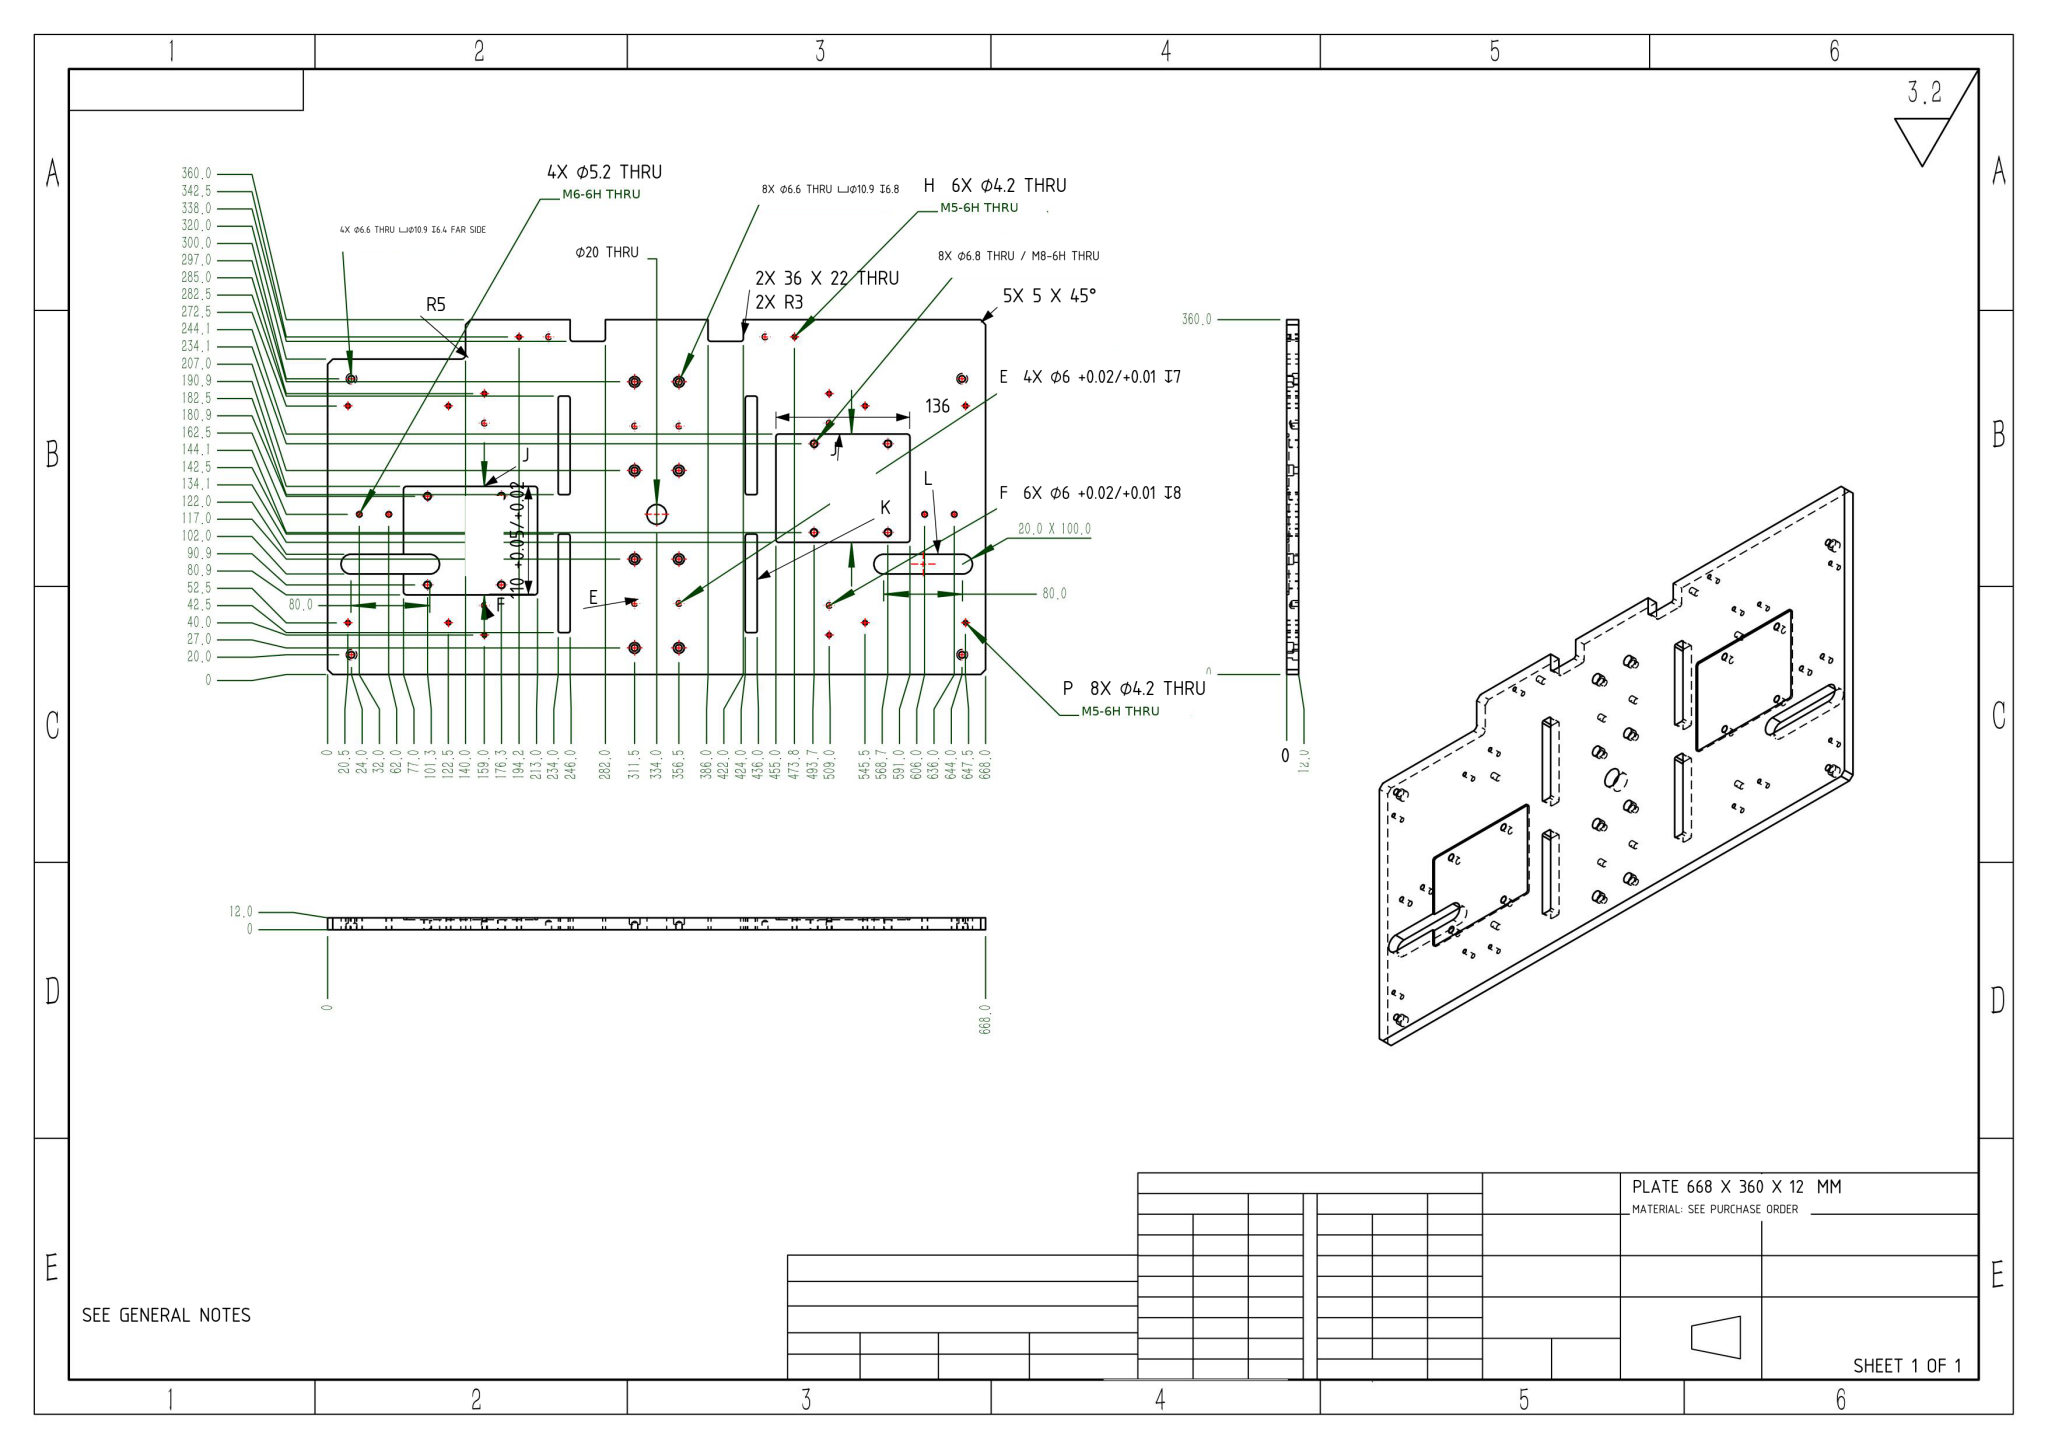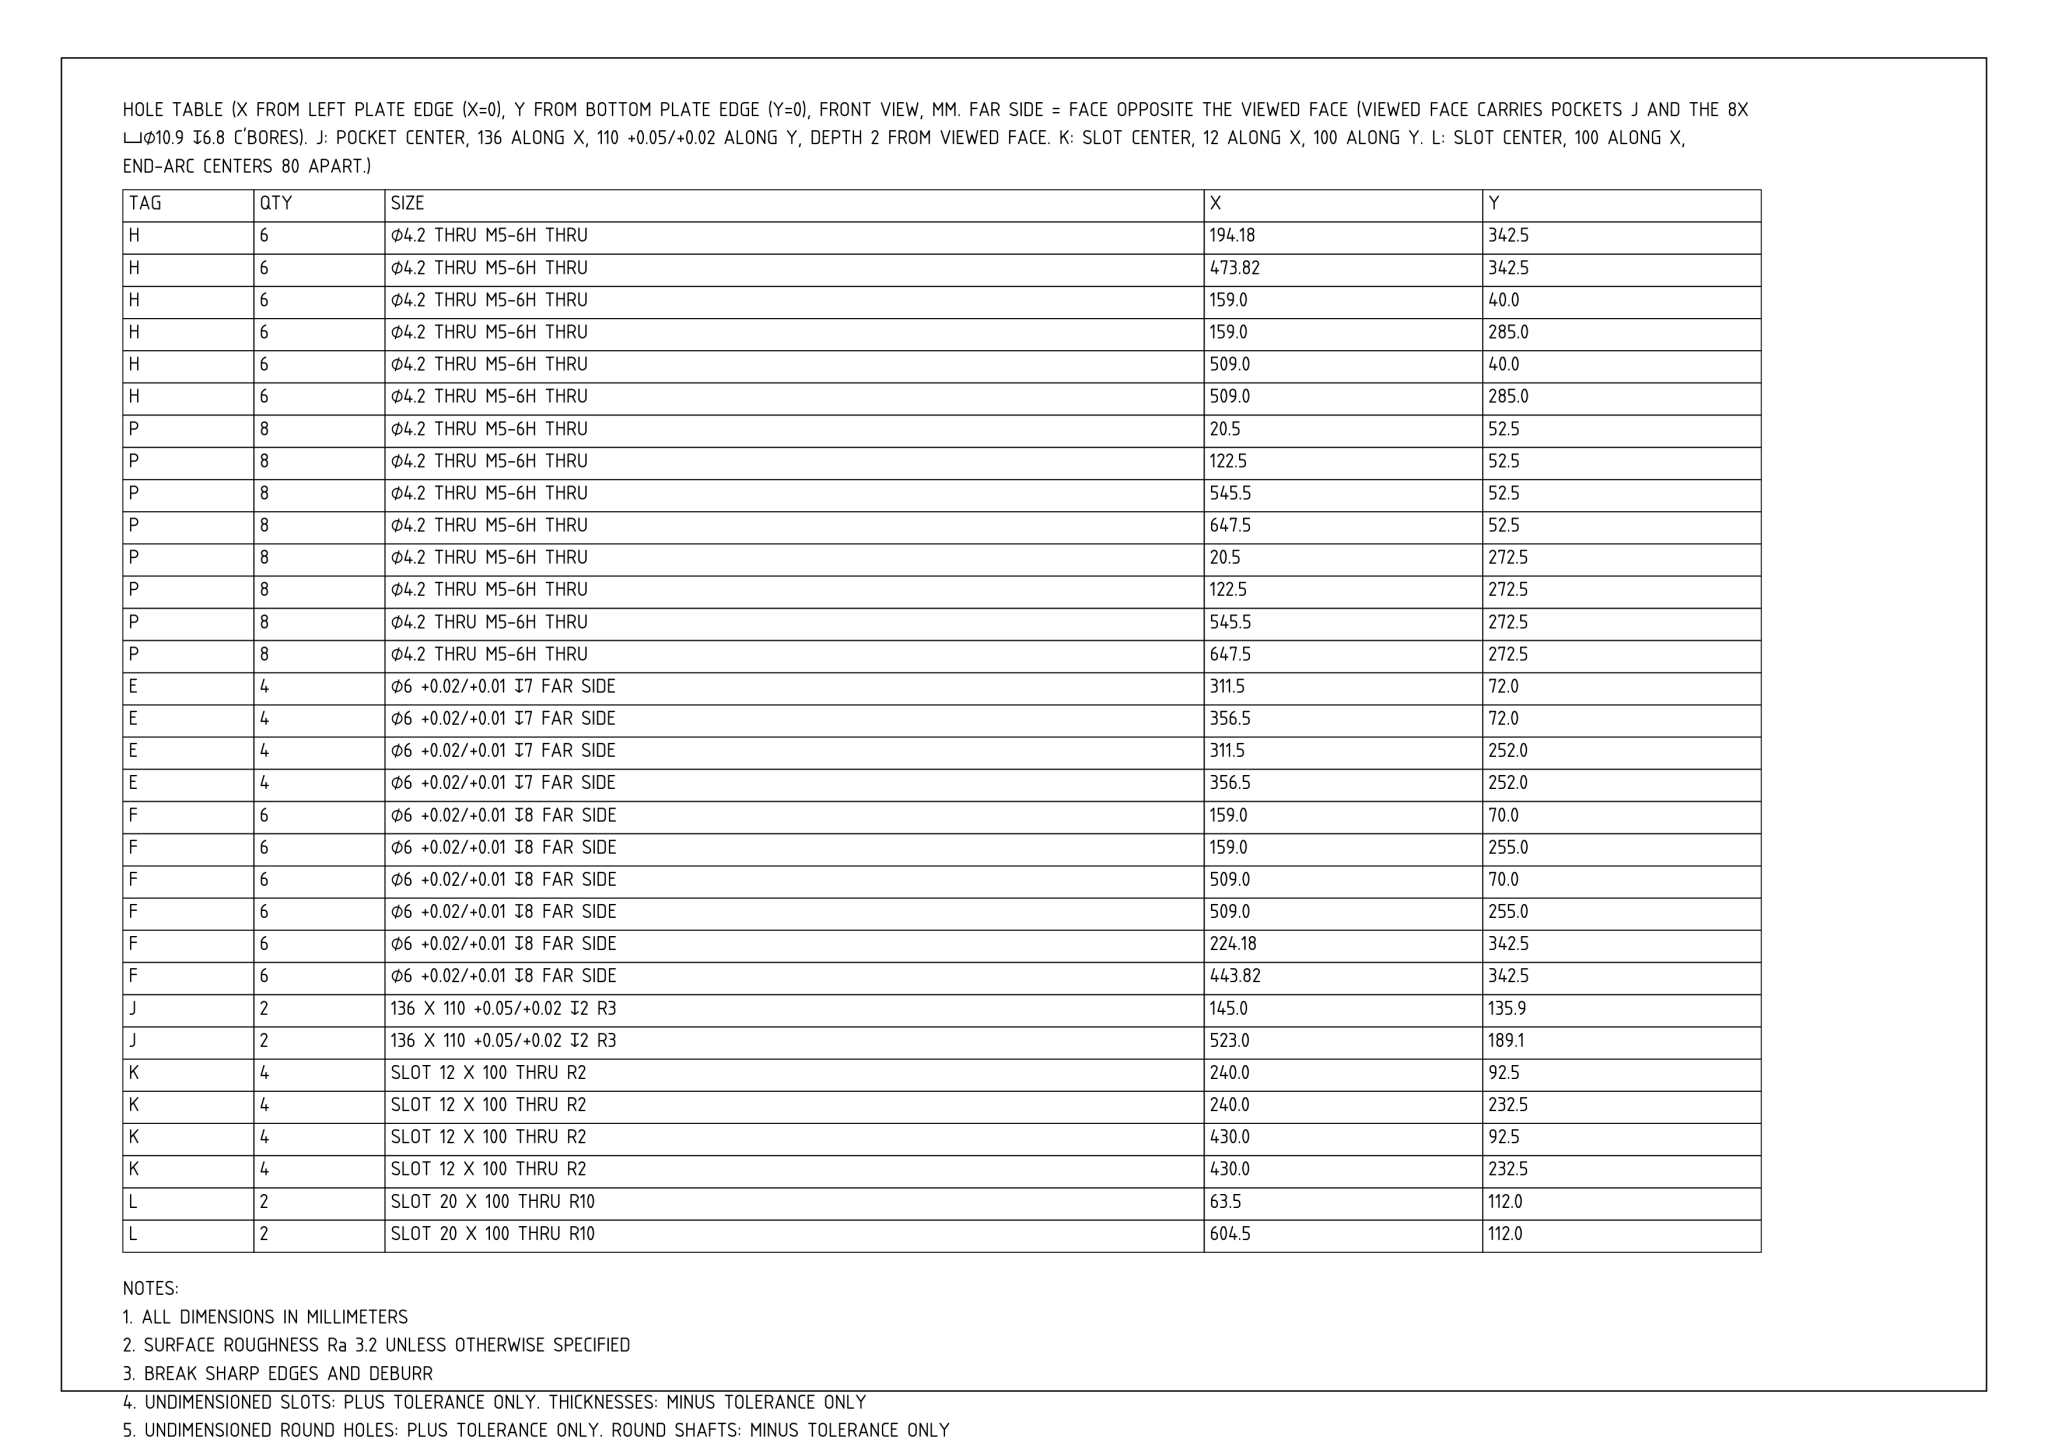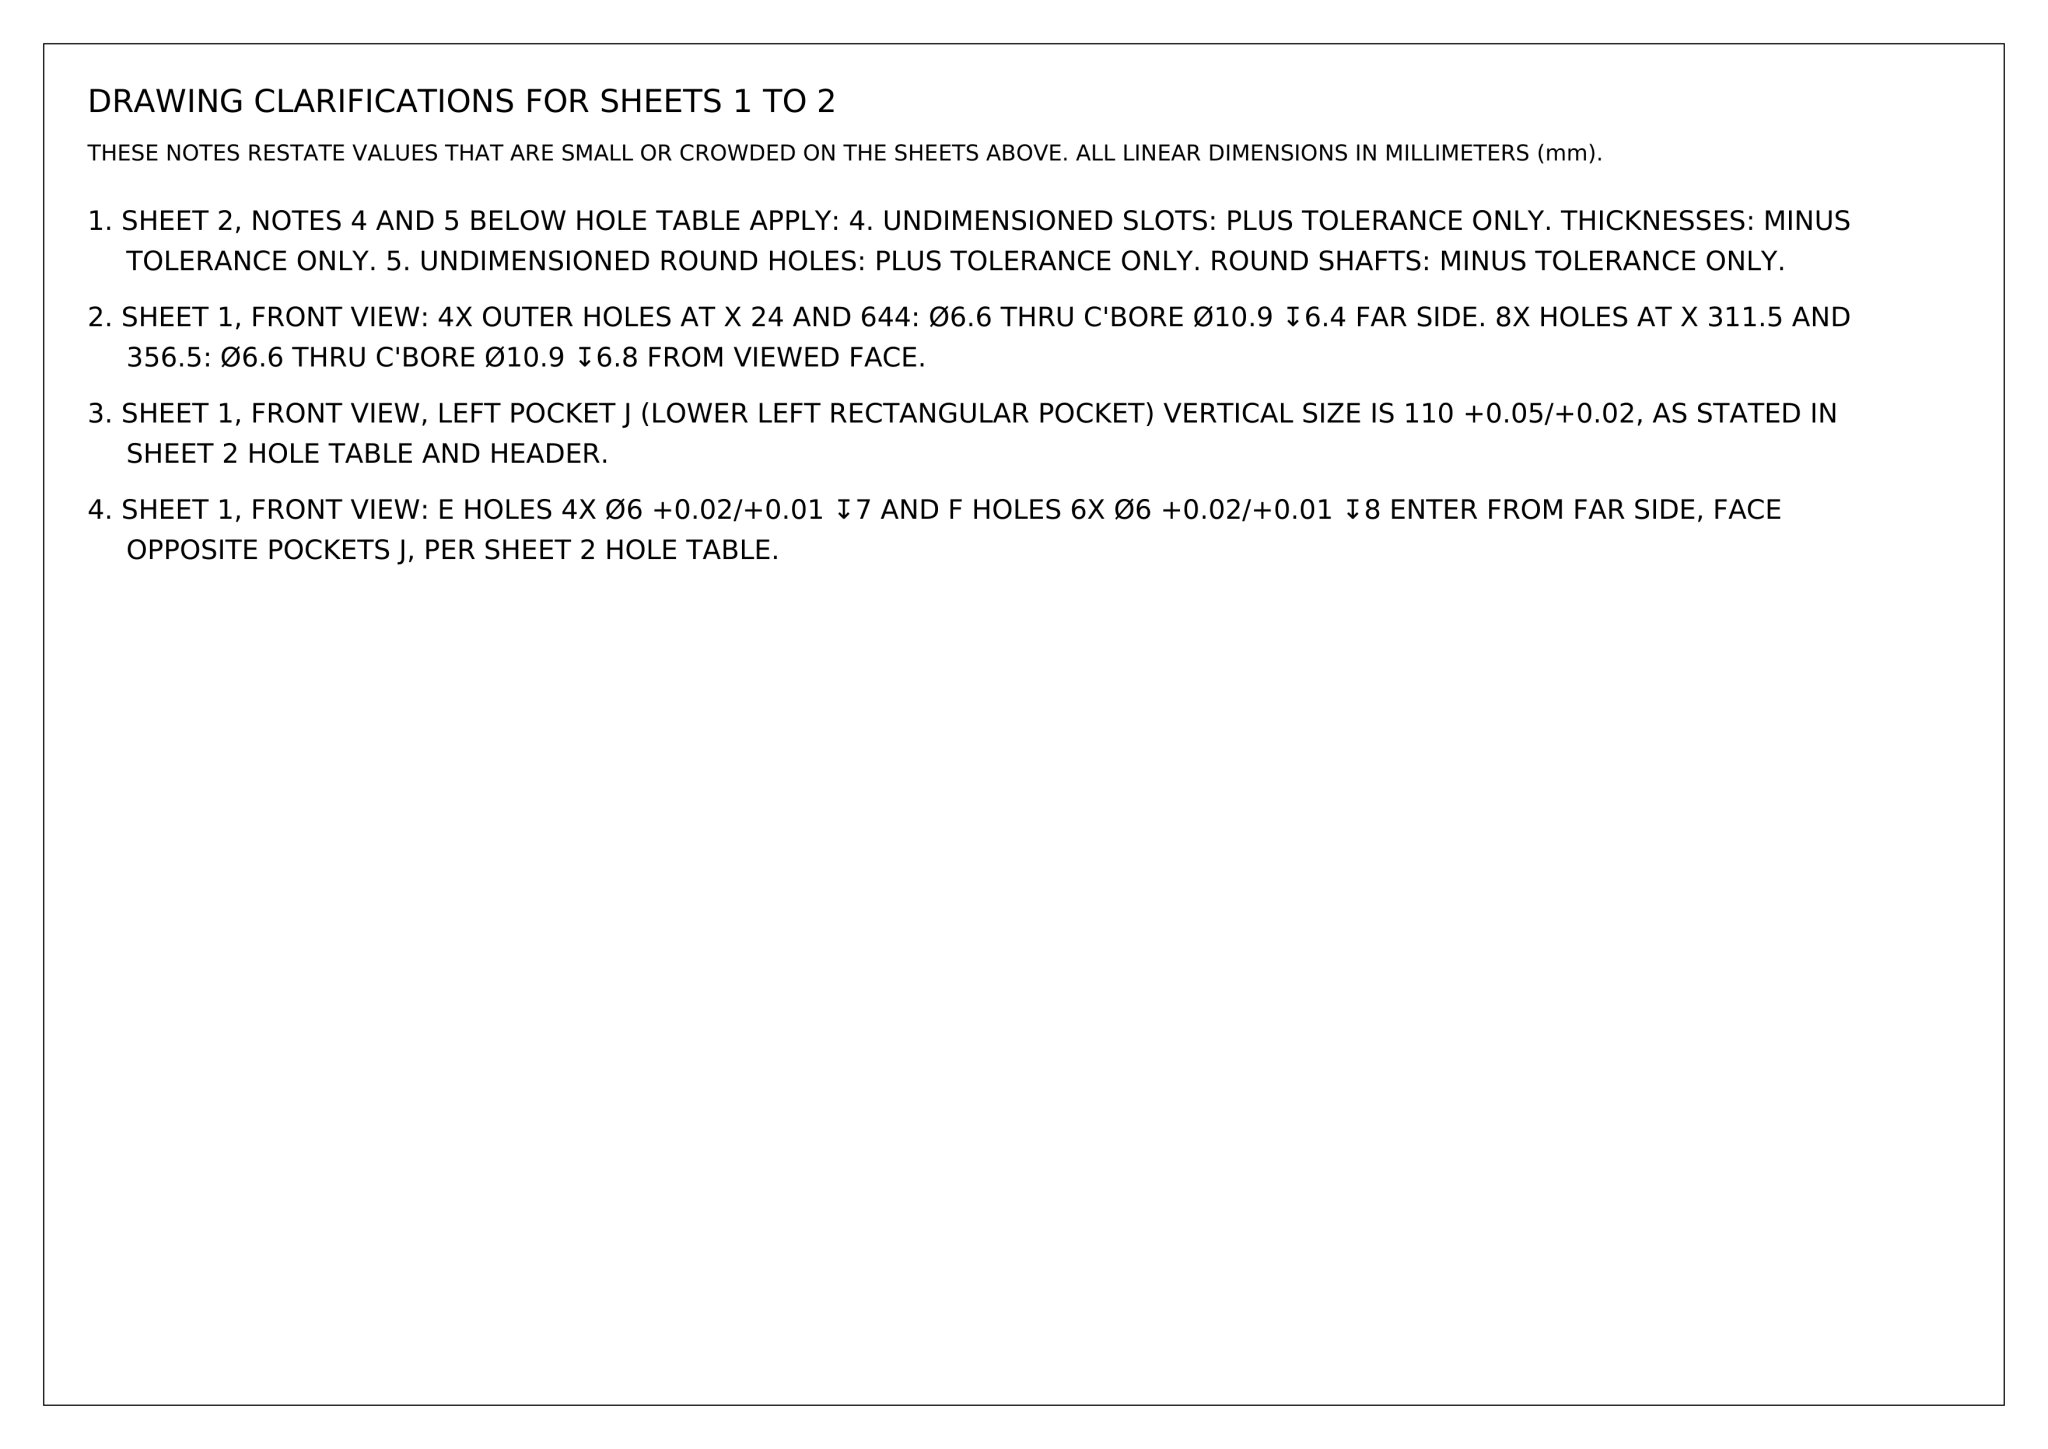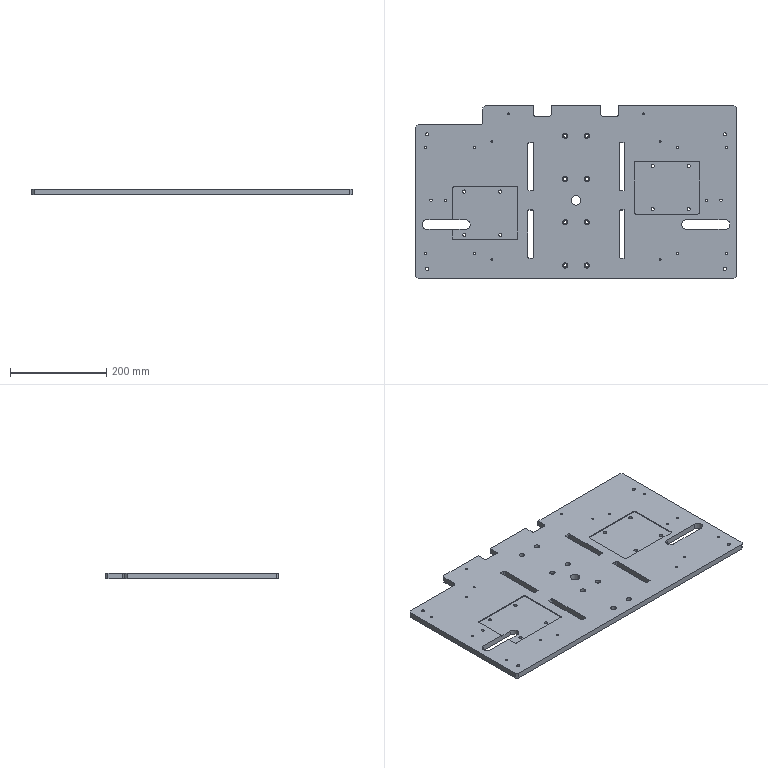Part | NX | mm | 1 solid | 241 faces | box 668 x 360 x 12 mm | volume 2615154 mm3 | cylinder 157 | plane 64 | cone 20 | commonest cylinder face diameters 6 x32 4.2 x28 10.9 x24 6.6 x24 6.8 x16 4 x16 5.2 x8 20 x8